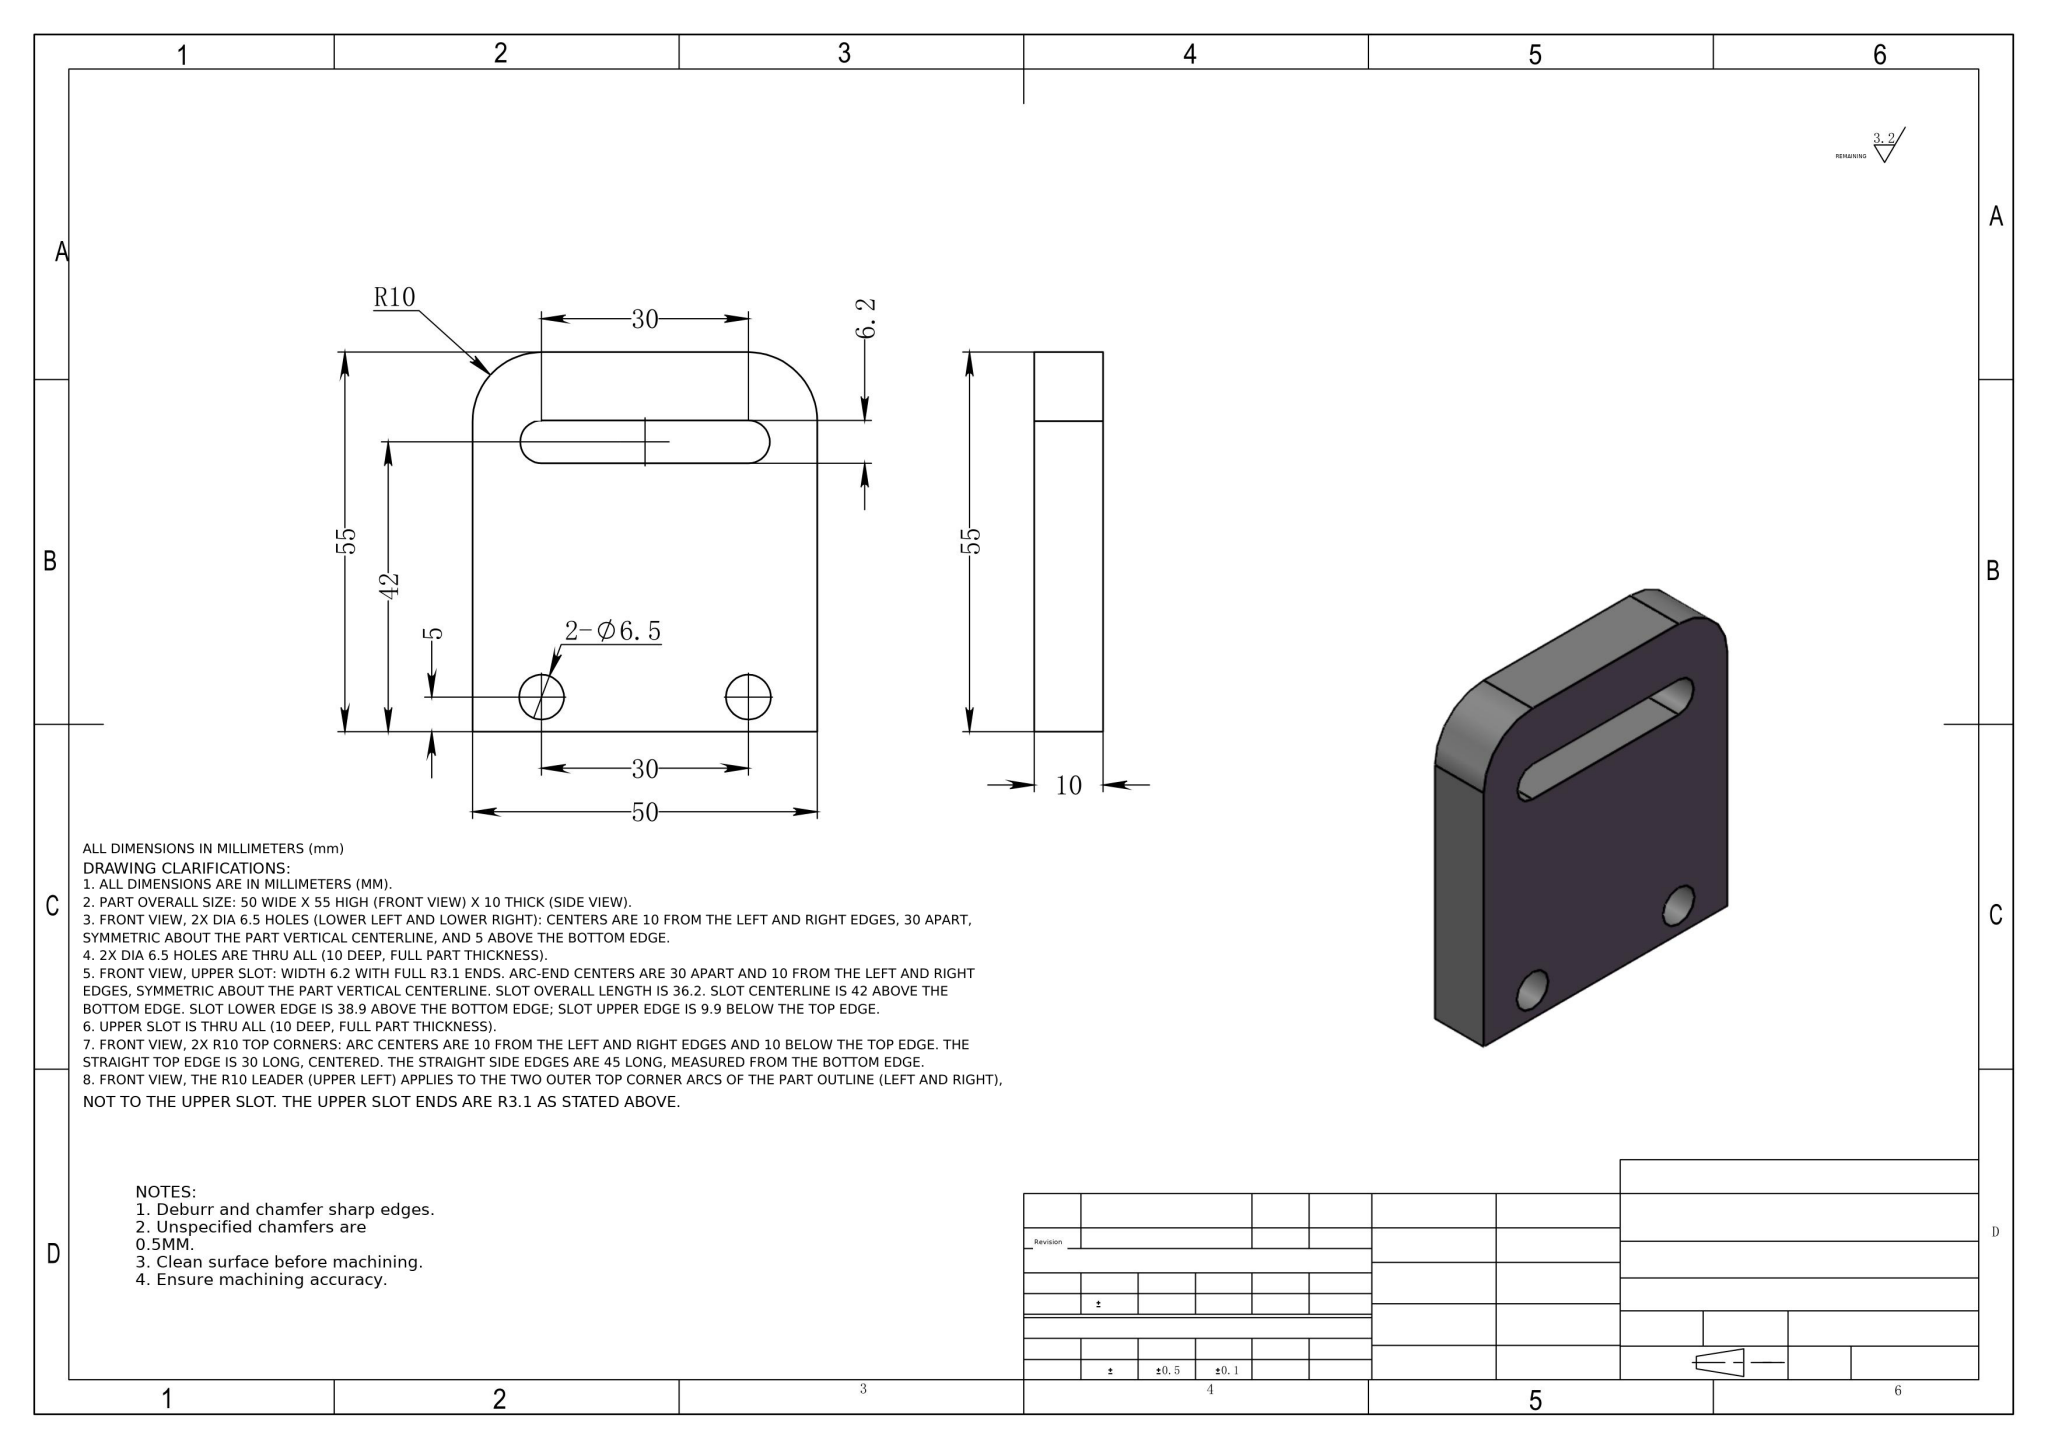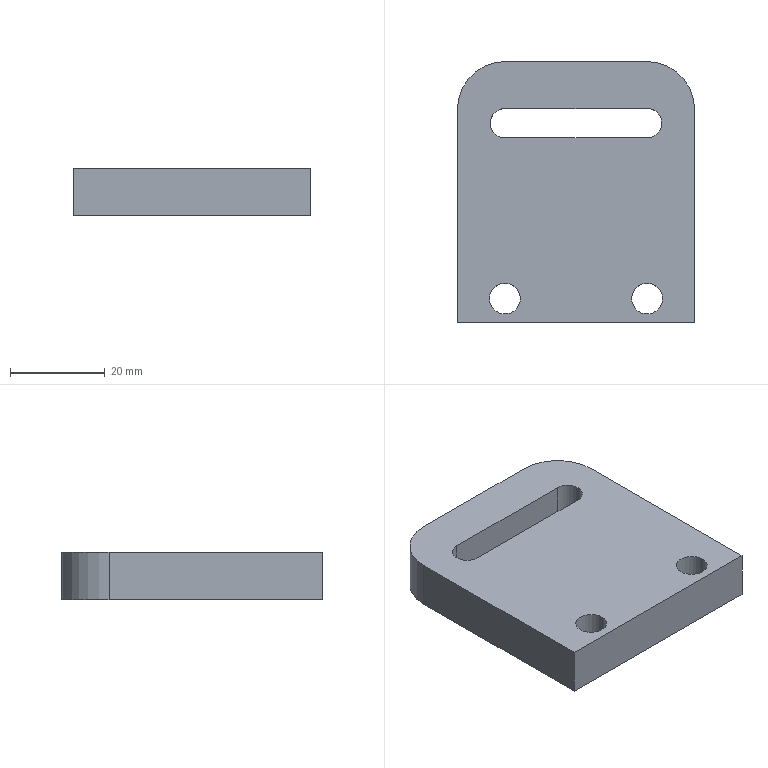Part | NX | mm | Rounded Corner Slotted Base Plate | 1 solid | 17 faces | box 50 x 55 x 10 mm | volume 24245 mm3 | cylinder 9 | plane 8 | commonest cylinder face diameters 6.5 x4 6.2 x3 20 x2